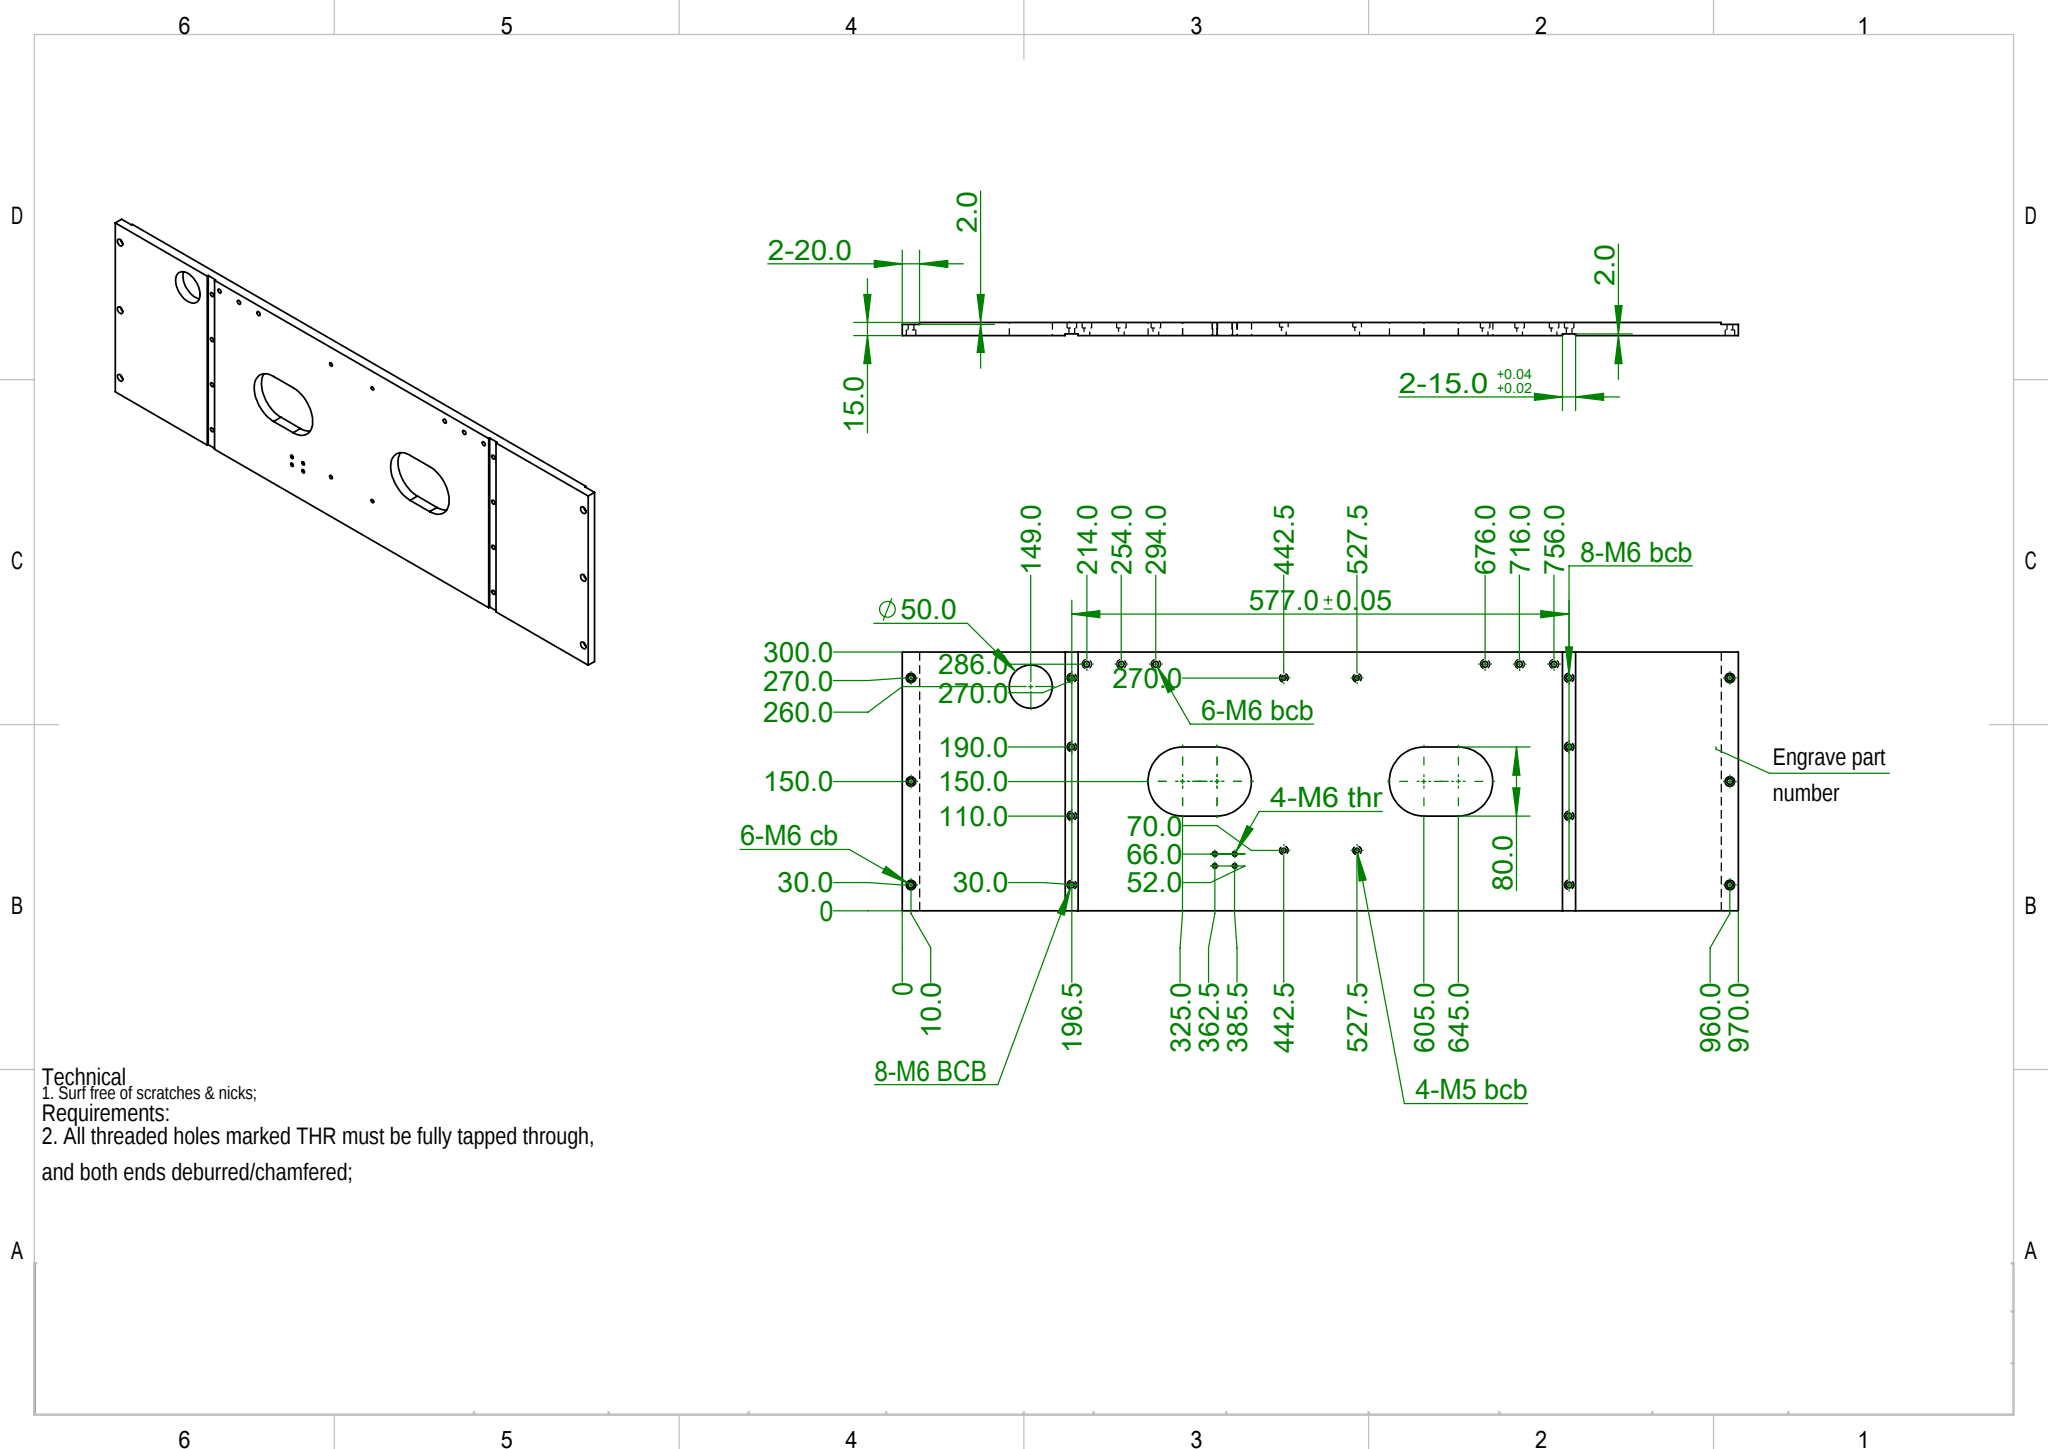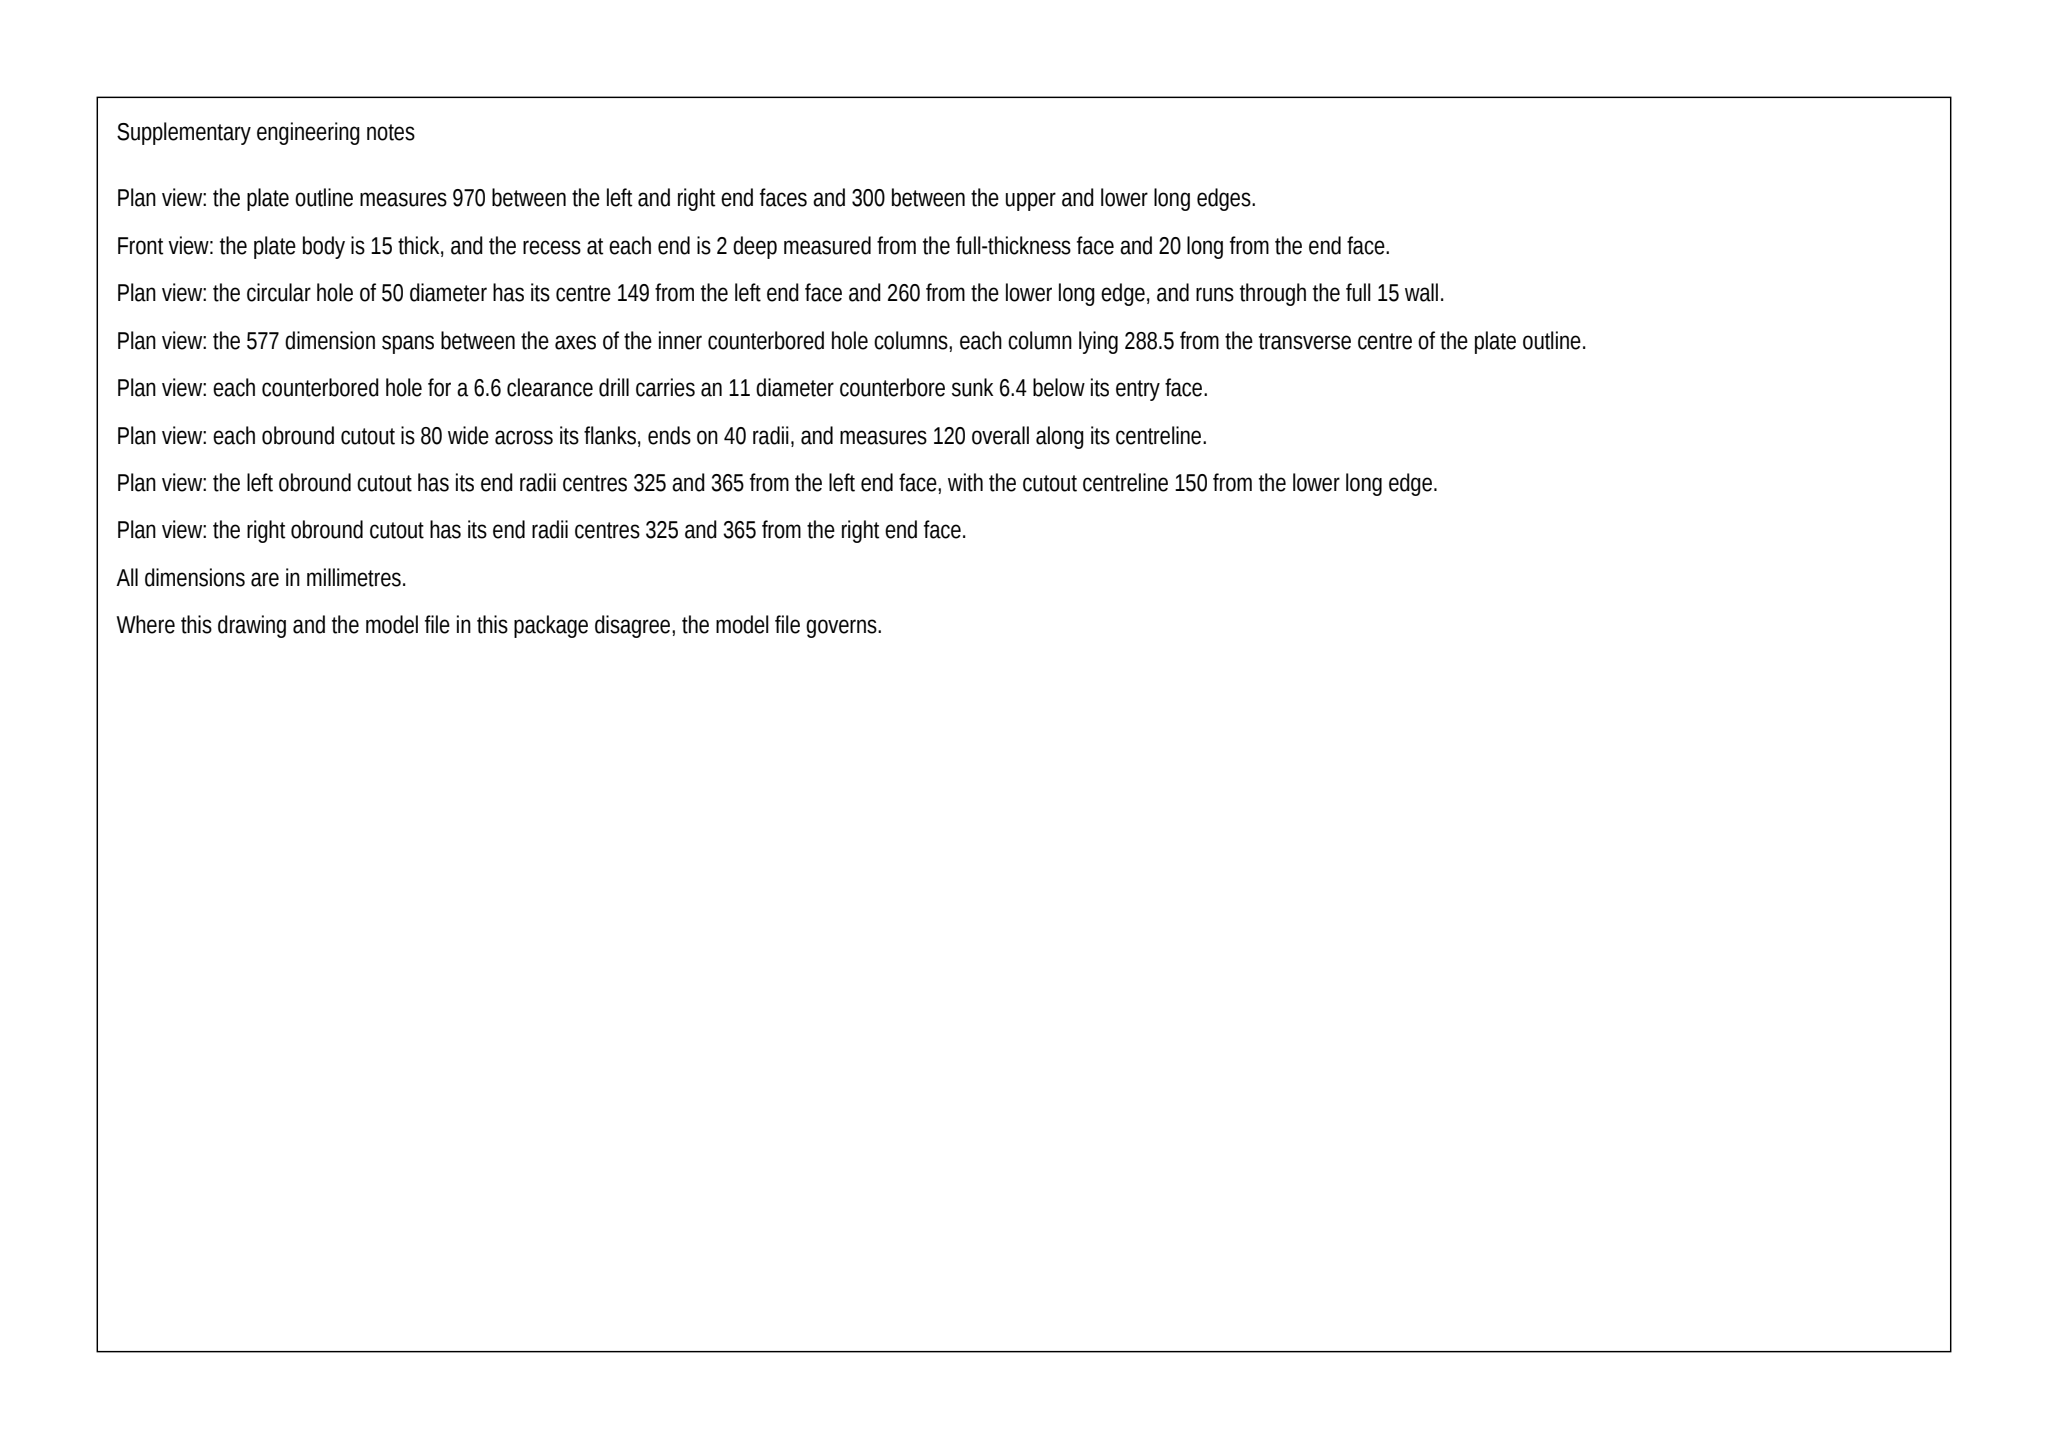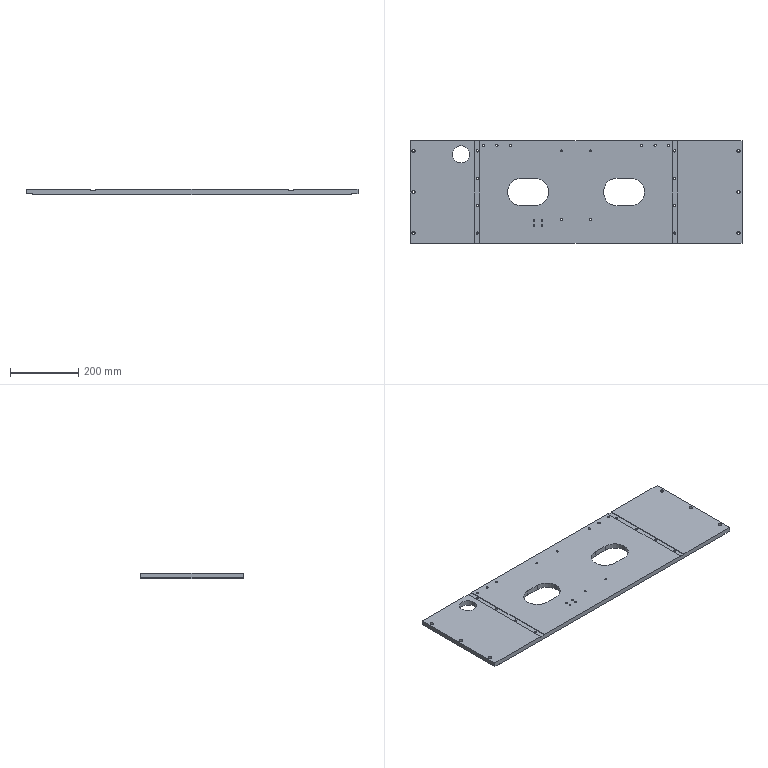Part | SolidWorks | mm | 1 solid | 182 faces | box 970 x 300 x 15 mm | volume 4025873 mm3 | cylinder 112 | plane 46 | cone 24 | commonest cylinder face diameters 11 x40 6.6 x40 5 x8 10 x8 5.5 x8 80 x6 50 x2
Drawing notes:
LH OBROUND SLOT: 2ND ARC CTR X=365.0, 40.0 BETWEEN CTRS | from the solid: cyl Ø80 z at [325.0,150.0] and [365.0,150.0], len 15.0 (LH slot)
LH SLOT WIDTH 80.0 TYP, SAME AS RH SLOT | from the solid: Ø80 end radii on both slots: [325/365,150] and [605/645,150]
2-15.0 WIDE x 2.0 DP STEPS AT X=189.0 & X=766.0 FROM LH END | from the solid: x-planes at 189.0/204.0 and 766.0/781.0; z-plane 13.0 (15.0-2.0)
ALL M6 cb/bcb: Ø6.6 THRU, Ø11.0 C'BORE DP 6.4 | from the solid: Ø6.6 holes len 6.6/8.6 + Ø11.0 len 6.38-6.4 (sum = local thk 13.0/15.0)
4-M5 bcb: Ø5.5 THRU, Ø10.0 C'BORE DP 5.4 | from the solid: Ø5.5 len 9.6 + Ø10.0 len 5.38 at [442.5/527.5, 70/270] = 15.0 thk
C'BORE MOUTHS C/SINK 90°: Ø11.05 (M6), Ø10.05 (M5) | from the solid: cones 90° ref dia 11.05 x16, 90° ref dia 10.05 x8
4-M6 thr: TAP THRU 15.0 (Ø5.0 DRILL), CLEAN CORNERS BOTH ENDS | from the solid: Ø5.0 z holes len 15.0 at [362.5/385.5, 52.0/66.0] = full thk
RH SLOT (R40 ARC CTRS X605.0/X645.0) CL AT Y150.0 FROM BTM EDGE | from the solid: 80 dia cyls z-axis at [605,150] and [645,150], bbox Y=300
6-M6 cb AT X10.0 & X960.0: C'BORE Ø11.0 DP 6.4 BOTH FACES | from the solid: Ø11.0 x 6.4 deep cbores, count 2 each at (10,30/150/270) & (960,30/150/270)